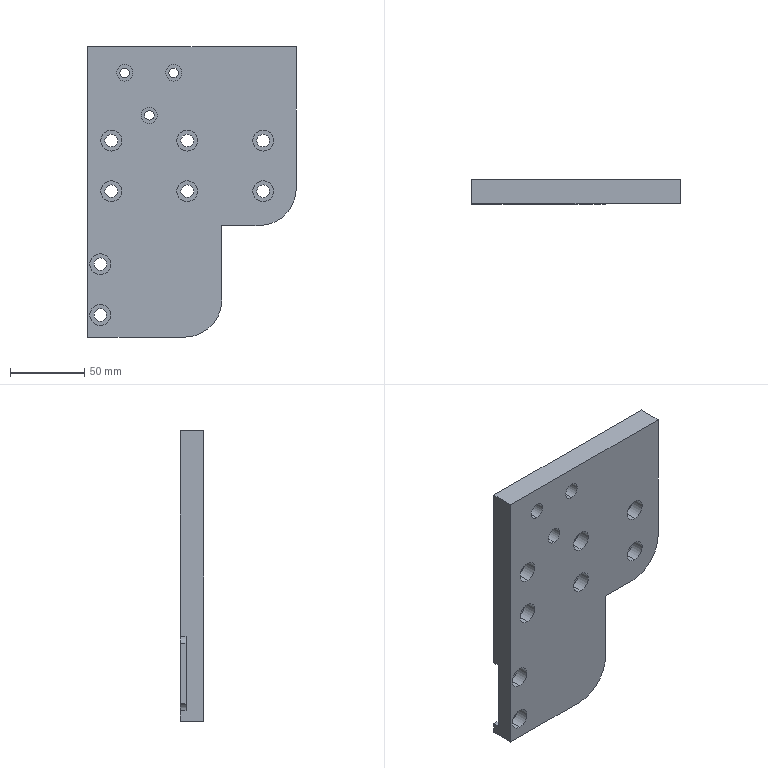Component | SolidWorks | BasePlate-1 | 1 solid | 114 faces | box 140 x 16 x 195 mm | volume 328288 mm3 | cylinder 74 | plane 40 | commonest cylinder face diameters 10 x24 14 x16 8.5 x16 11 x6 6.5 x6 45 x4 50 x2
build123d program:
from build123d import *

# Parameters (mm, degrees)
BOSS_EXTRUDE1_DEPTH                                  = 16
CUT_EXTRUDE1_DEPTH                                   = 4
HOLE_SIZE_ACCORDING_TO_HEXAGON_SOCKET_HE_D           = 8.5
HOLE_SIZE_ACCORDING_TO_HEXAGON_SOCKET_HE_CBORE_D     = 14
HOLE_SIZE_ACCORDING_TO_HEXAGON_SOCKET_HE_CBORE_DEPTH = 9
SKETCH14_W                                           = 120
SKETCH14_H                                           = 50
BOSS_EXTRUDE2_DEPTH                                  = 16
CUT_EXTRUDE2_DEPTH                                   = 4
HOLE_SIZE_ACCORDING_TO_HEXAGON_SOCKE_2_D             = 8.5
HOLE_SIZE_ACCORDING_TO_HEXAGON_SOCKE_2_CBORE_D       = 14
HOLE_SIZE_ACCORDING_TO_HEXAGON_SOCKE_2_CBORE_DEPTH   = 9
SKETCH10_R                                           = 22.5
CUT_EXTRUDE3_DEPTH                                   = 4
FILLET1_R                                            = 25
HOLE_SIZE_ACCORDING_TO_HEXAGON_SOCKE_3_D             = 6.5
HOLE_SIZE_ACCORDING_TO_HEXAGON_SOCKE_3_CBORE_D       = 11
HOLE_SIZE_ACCORDING_TO_HEXAGON_SOCKE_3_CBORE_DEPTH   = 8


with BuildPart() as part:
    # Sketch1 → Boss-Extrude1 (new body)
    with BuildSketch(Plane.XY):
        with BuildLine():
            Line((-97.5, 45), (72.5, 45))
            ThreePointArc((72.5, 45), (90.178, 37.678), (97.5, 20))
            Line((97.5, 20), (97.5, -45))
            Line((97.5, -45), (-97.5, -45))
            Line((-97.5, -45), (-97.5, 45))
        make_face()
    extrude(amount=BOSS_EXTRUDE1_DEPTH)

    # Sketch2 → Cut-Extrude1 (cut)
    with BuildSketch(Plane.XY):
        with BuildLine():
            Line((90.5, -45), (90.5, -28.118))
            ThreePointArc((90.5, -28.118), (93.292, -18.97), (85.868, -25))
            Line((85.868, -25), (45.132, -25))
            ThreePointArc((45.132, -25), (37.708, -18.97), (40.5, -28.118))
            Line((40.5, -28.118), (40.5, -45))
            Line((40.5, -45), (90.5, -45))
        make_face()
    extrude(amount=CUT_EXTRUDE1_DEPTH, mode=Mode.SUBTRACT)

    # Hole Size_according to_Hexagon Socket He (through all)
    with Locations(Plane(origin=(0, 0, 16), x_dir=(-1, 0, 0), z_dir=(0, 0, 1))):
        with Locations((-48.5, 36.559), (-82.5, 36.559)):
            CounterBoreHole(HOLE_SIZE_ACCORDING_TO_HEXAGON_SOCKET_HE_D / 2, HOLE_SIZE_ACCORDING_TO_HEXAGON_SOCKET_HE_CBORE_D / 2, HOLE_SIZE_ACCORDING_TO_HEXAGON_SOCKET_HE_CBORE_DEPTH)

    # Sketch14 → Boss-Extrude2 (add)
    with BuildSketch(Plane(origin=(0, 0, 0), x_dir=(-1, 0, 0), z_dir=(0, 0, -1))):
        with Locations((37.5, 70)):
            Rectangle(SKETCH14_W, SKETCH14_H)
    extrude(amount=-BOSS_EXTRUDE2_DEPTH)

    # Sketch6 → Cut-Extrude2 (cut)
    with BuildSketch(Plane.XY):
        with BuildLine():
            Line((-37.5, -36.7), (2.5, -36.7))
            ThreePointArc((2.5, -36.7), (11.036, -40.236), (7.5, -31.7))
            Line((7.5, -31.7), (7.5, -26.7))
            ThreePointArc((7.5, -26.7), (11.036, -18.164), (2.5, -21.7))
            Line((2.5, -21.7), (-37.5, -21.7))
            ThreePointArc((-37.5, -21.7), (-46.036, -18.164), (-42.5, -26.7))
            Line((-42.5, -26.7), (-42.5, -31.7))
            ThreePointArc((-42.5, -31.7), (-46.036, -40.236), (-37.5, -36.7))
        make_face()
        with BuildLine():
            Line((-37.5, 80.3), (2.5, 80.3))
            ThreePointArc((2.5, 80.3), (11.036, 83.836), (7.5, 75.3))
            Line((7.5, 75.3), (7.5, 70.3))
            ThreePointArc((7.5, 70.3), (11.036, 61.764), (2.5, 65.3))
            Line((2.5, 65.3), (-37.5, 65.3))
            ThreePointArc((-37.5, 65.3), (-46.036, 61.764), (-42.5, 70.3))
            Line((-42.5, 70.3), (-42.5, 75.3))
            ThreePointArc((-42.5, 75.3), (-46.036, 83.836), (-37.5, 80.3))
        make_face()
        with BuildLine():
            Line((-37.5, 29.3), (2.5, 29.3))
            ThreePointArc((2.5, 29.3), (11.036, 32.836), (7.5, 24.3))
            Line((7.5, 24.3), (7.5, 19.3))
            ThreePointArc((7.5, 19.3), (11.036, 10.764), (2.5, 14.3))
            Line((2.5, 14.3), (-37.5, 14.3))
            ThreePointArc((-37.5, 14.3), (-46.036, 10.764), (-42.5, 19.3))
            Line((-42.5, 19.3), (-42.5, 24.3))
            ThreePointArc((-42.5, 24.3), (-46.036, 32.836), (-37.5, 29.3))
        make_face()
    extrude(amount=CUT_EXTRUDE2_DEPTH, mode=Mode.SUBTRACT)

    # Hole Size_according to_Hexagon Socke 2 (through all)
    with Locations(Plane(origin=(0, 0, 16), x_dir=(-1, 0, 0), z_dir=(0, 0, 1))):
        with Locations((34.5, -21.8), (0.5, -21.8), (0.5, 29.2), (34.5, 29.2), (0.5, -72.8), (34.5, -72.8)):
            CounterBoreHole(HOLE_SIZE_ACCORDING_TO_HEXAGON_SOCKE_2_D / 2, HOLE_SIZE_ACCORDING_TO_HEXAGON_SOCKE_2_CBORE_D / 2, HOLE_SIZE_ACCORDING_TO_HEXAGON_SOCKE_2_CBORE_DEPTH)

    # Sketch10 → Cut-Extrude3 (cut)
    with BuildSketch(Plane.XY):
        with Locations((-70.5, -3.7)):
            Circle(SKETCH10_R)
        with Locations((-70.5, 47.3)):
            Circle(SKETCH10_R)
    extrude(amount=CUT_EXTRUDE3_DEPTH, mode=Mode.SUBTRACT)

    # Fillet1
    fillet1_edges = [part.edges().sort_by_distance(p)[0] for p in [
        (22.5, 95, 8),
    ]]
    fillet(fillet1_edges, radius=FILLET1_R)

    # Hole Size_according to_Hexagon Socke 3 (through all)
    with Locations(Plane(origin=(0, 0, 16), x_dir=(-1, 0, 0), z_dir=(0, 0, 1))):
        with Locations((51.5, 3.7), (80, 20.154), (80, -12.754)):
            CounterBoreHole(HOLE_SIZE_ACCORDING_TO_HEXAGON_SOCKE_3_D / 2, HOLE_SIZE_ACCORDING_TO_HEXAGON_SOCKE_3_CBORE_D / 2, HOLE_SIZE_ACCORDING_TO_HEXAGON_SOCKE_3_CBORE_DEPTH)


solid = part.part

# Placed as in the assembly
solid = solid.moved(Location((115.246, 16, 421.171), (90, 0, -90)))